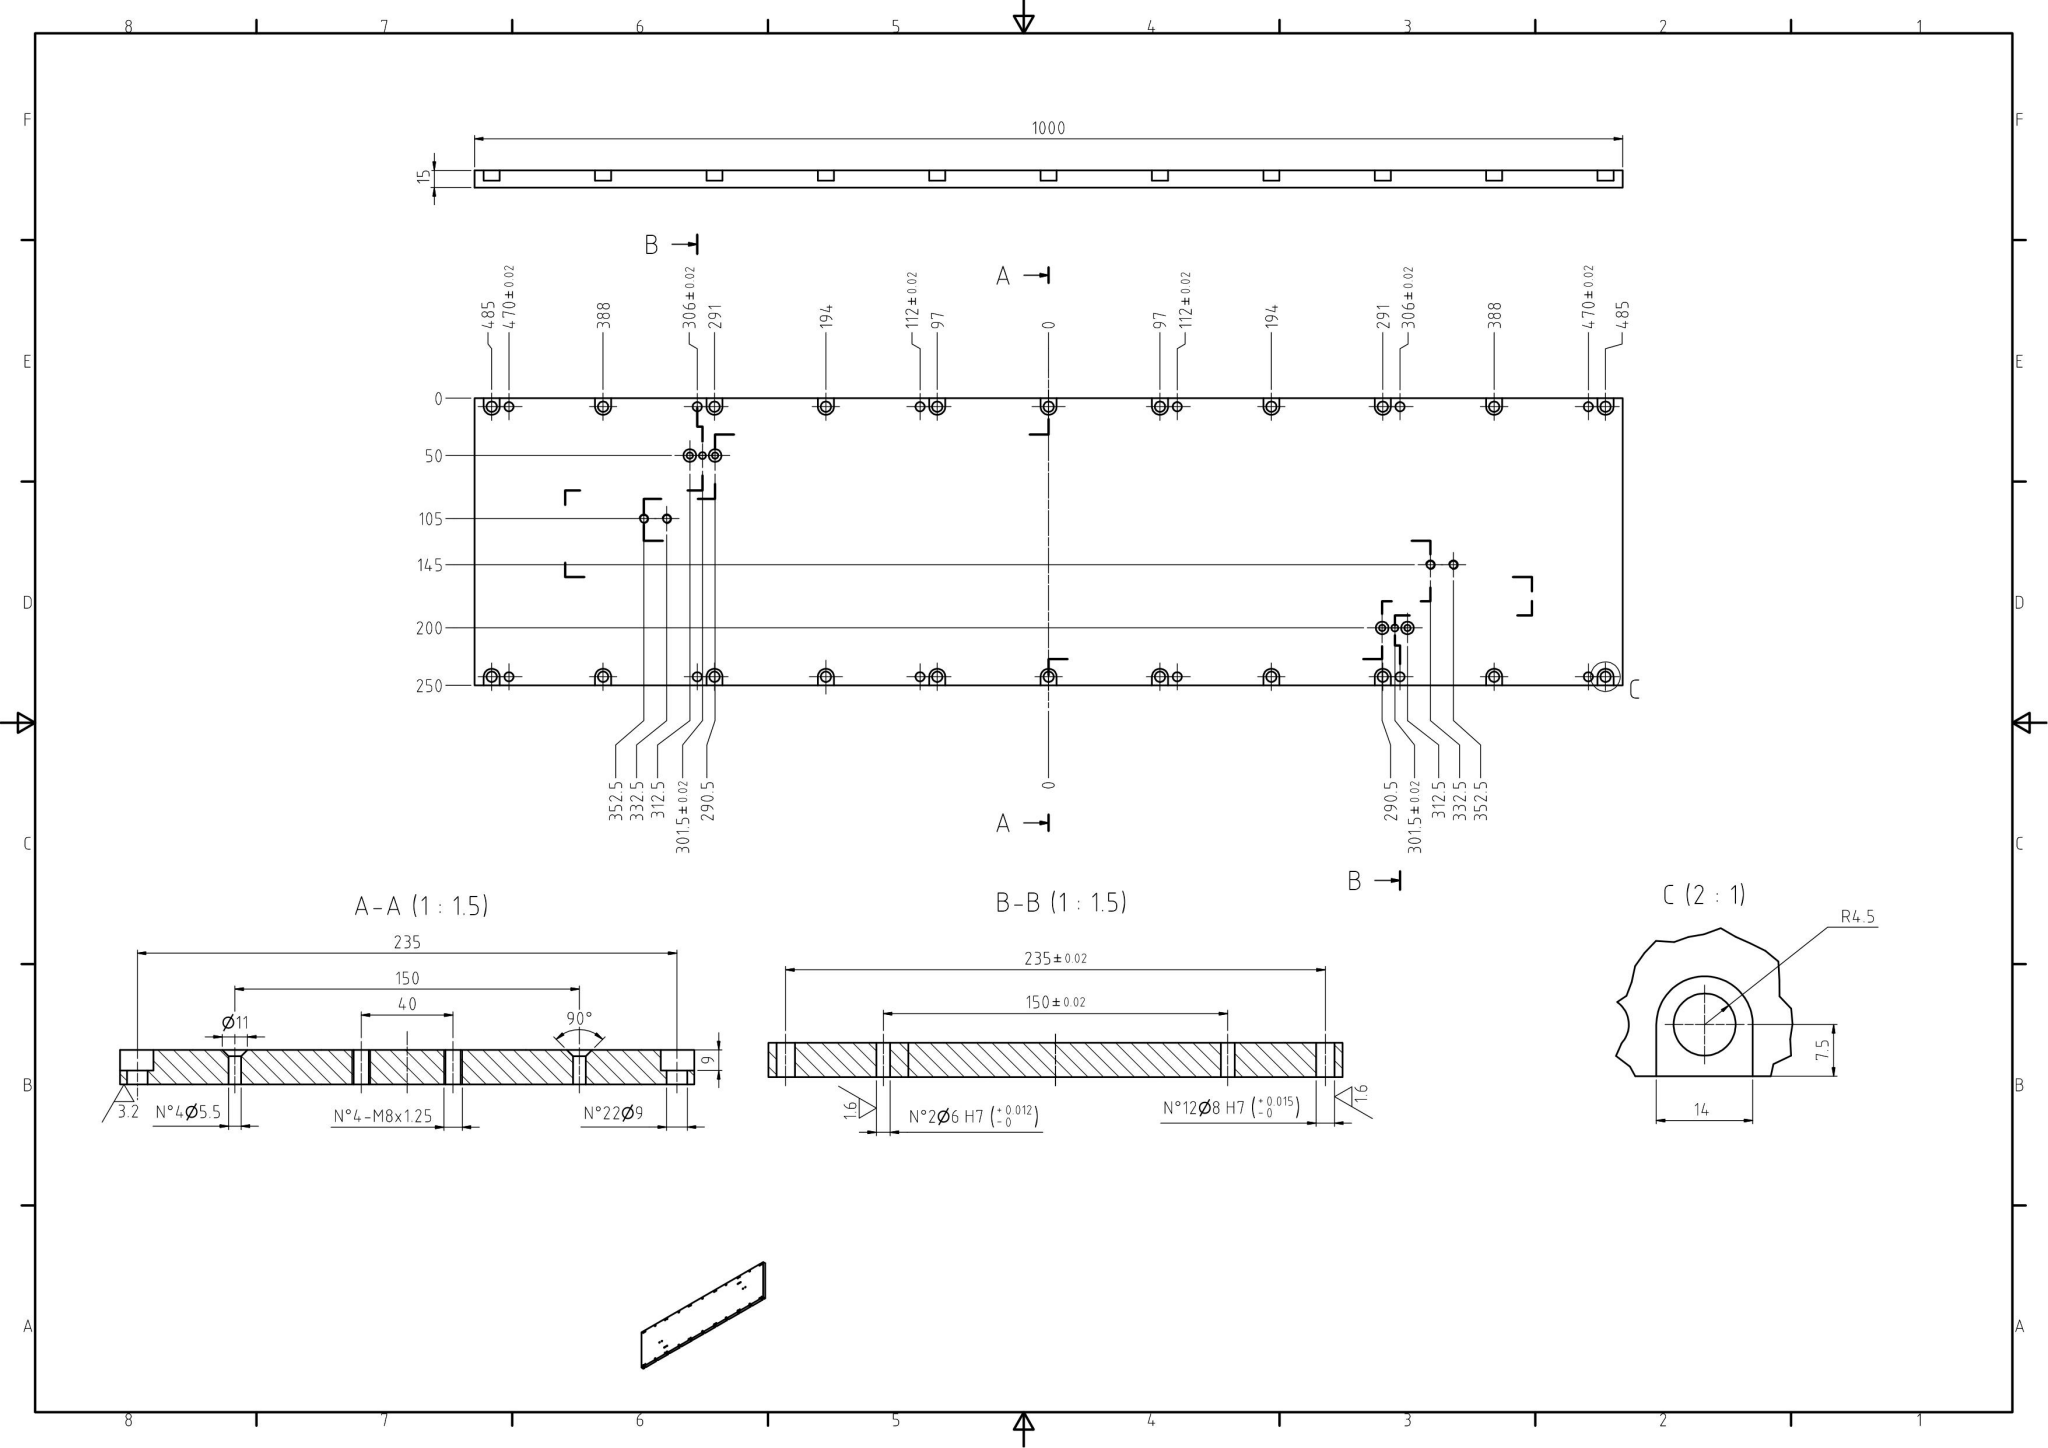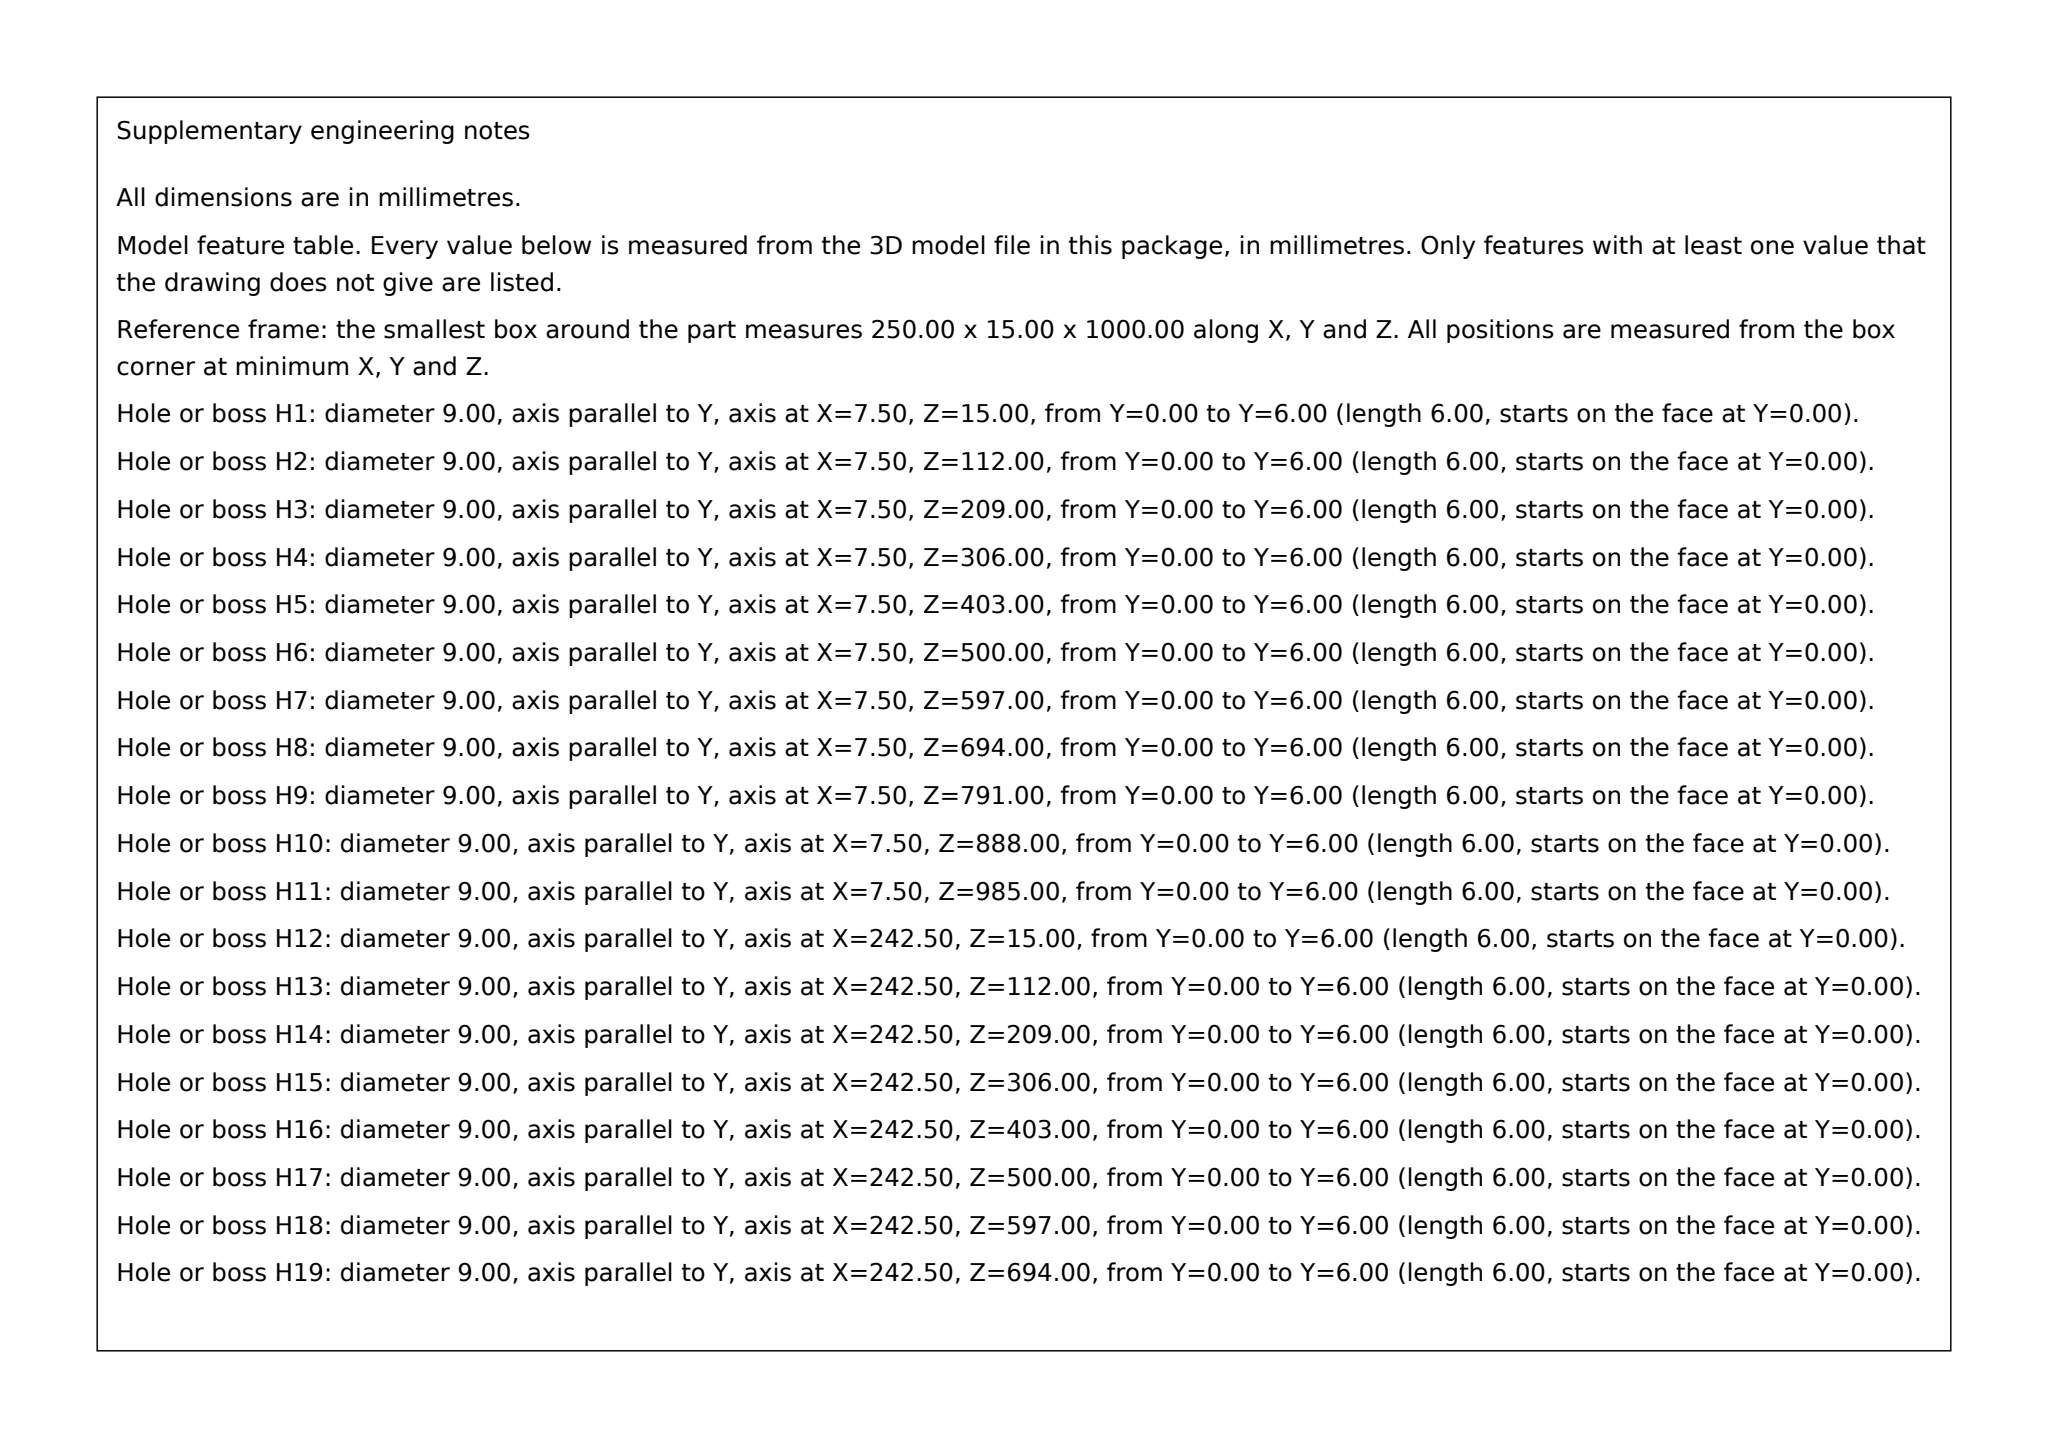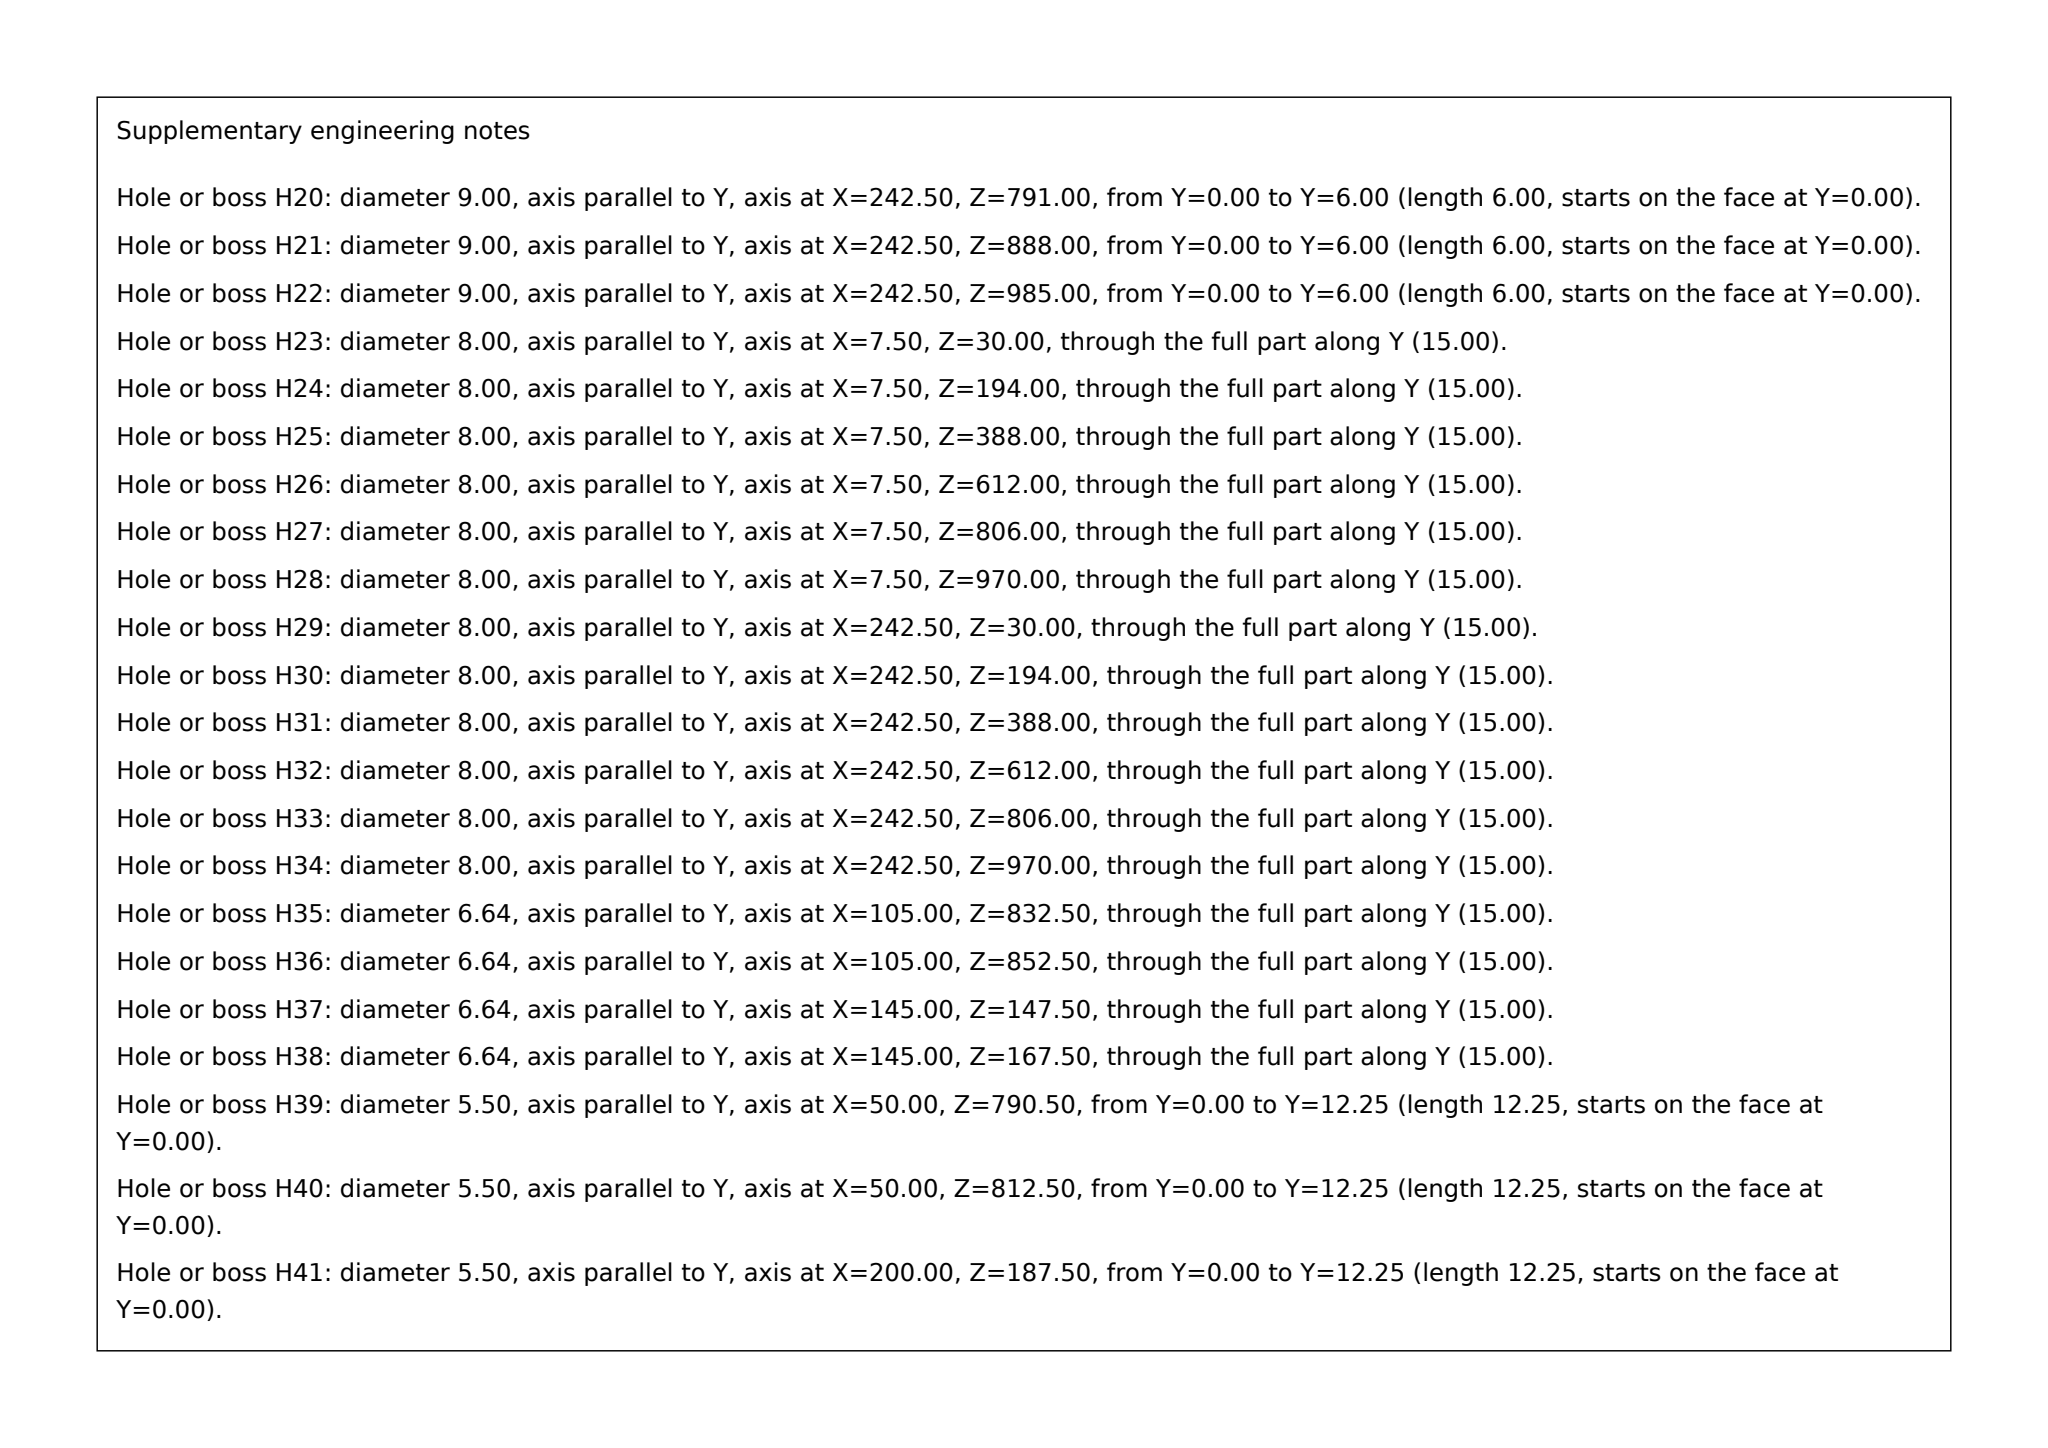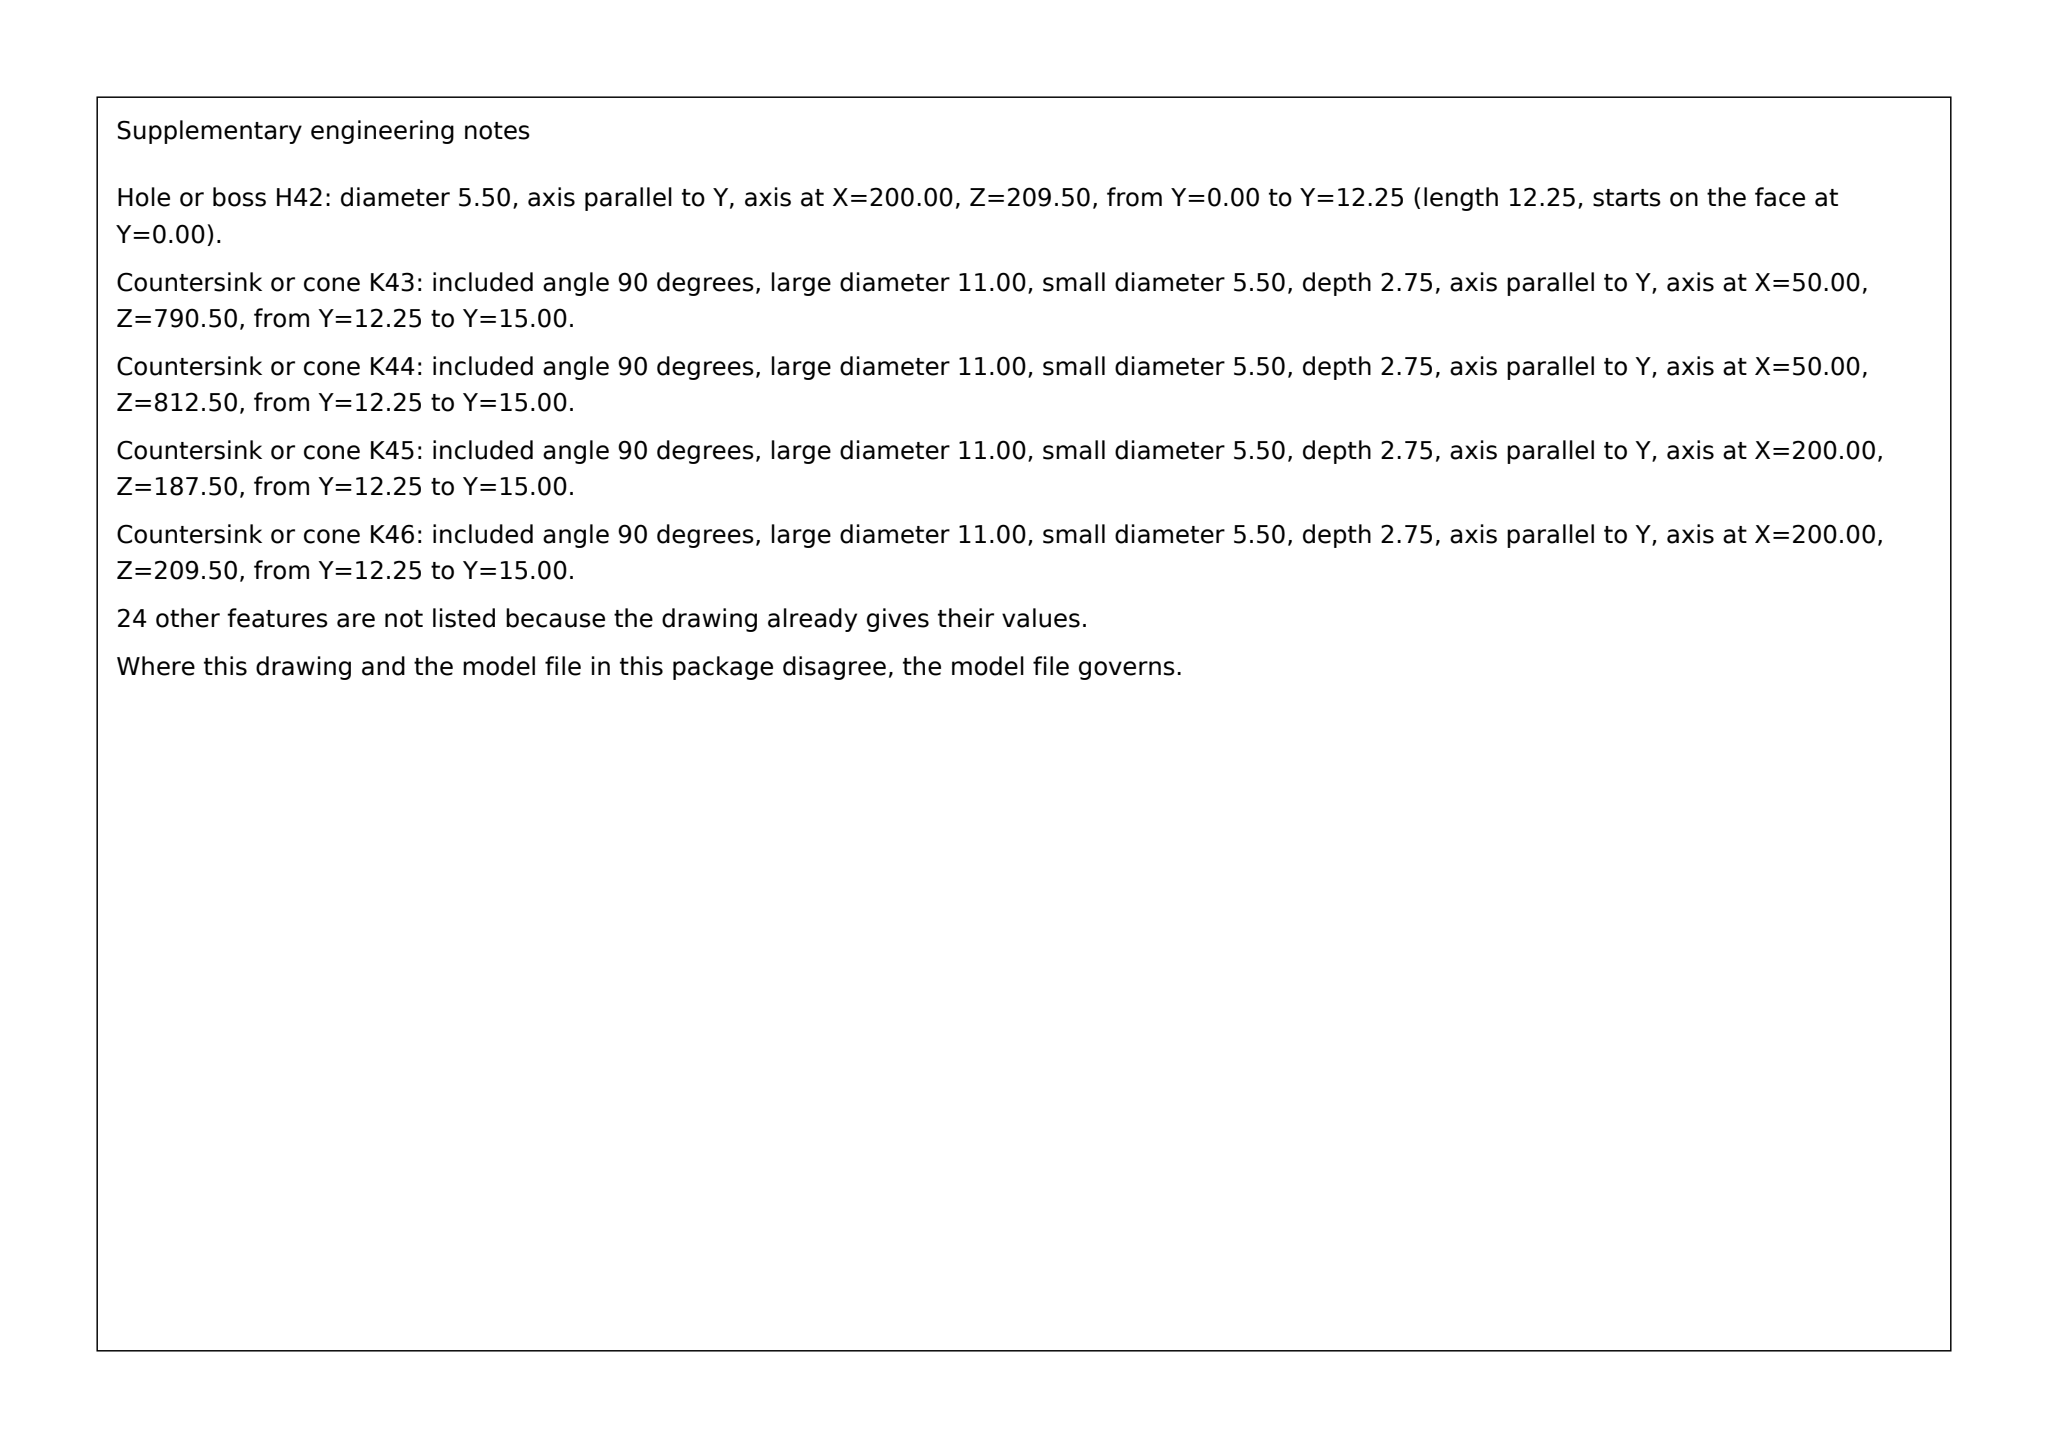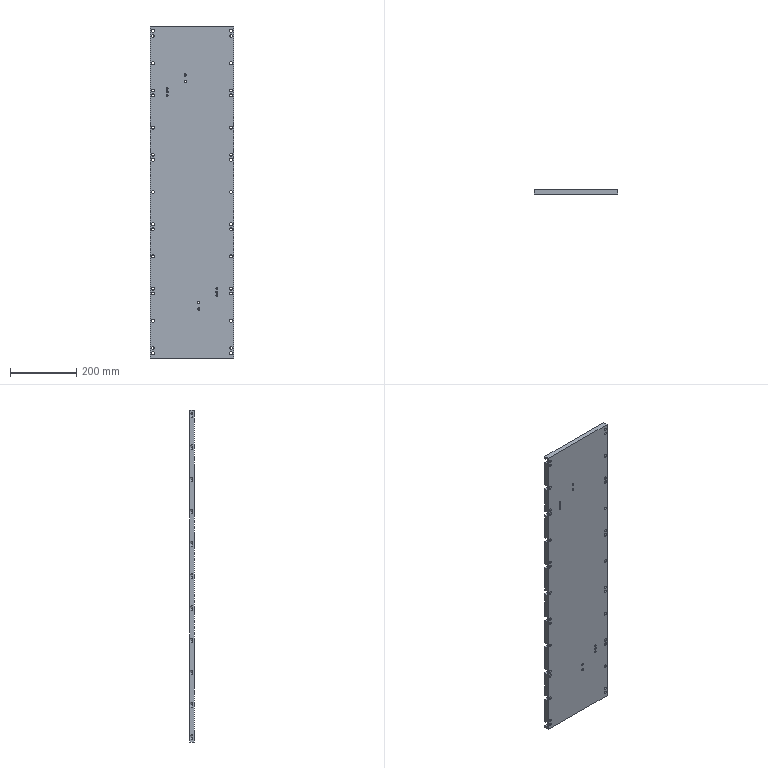Part | SolidWorks | mm | 1 solid | 212 faces | box 250 x 15 x 1000 mm | volume 3691821 mm3 | cylinder 132 | plane 72 | cone 8 | commonest cylinder face diameters 9 x44 14 x44 8 x24 5.5 x8 6.647 x8 6 x4